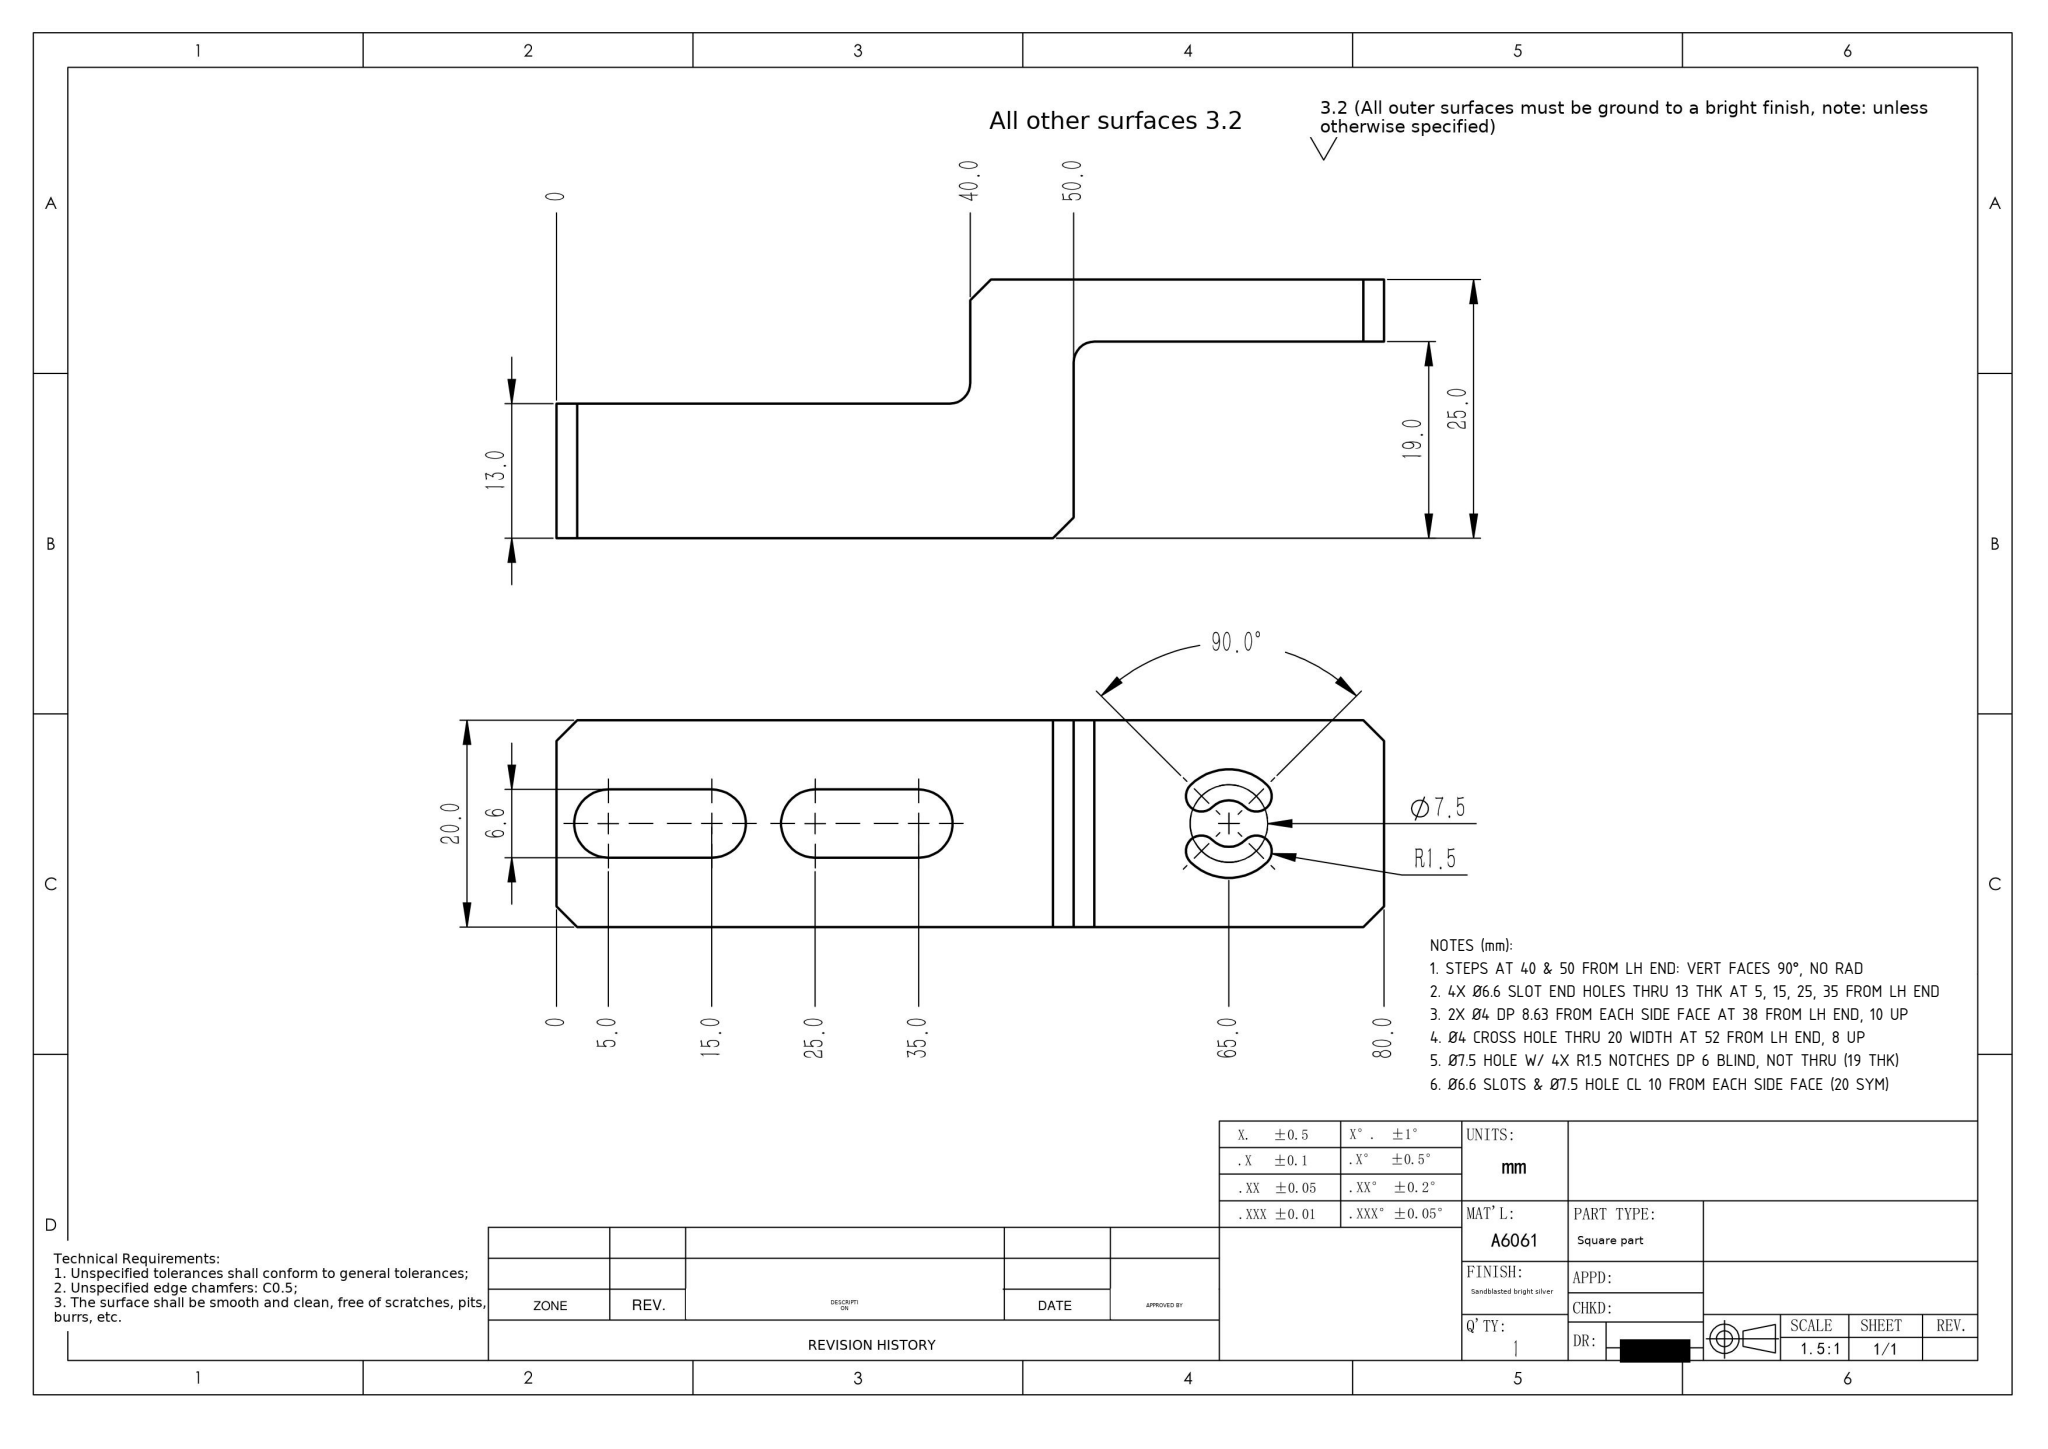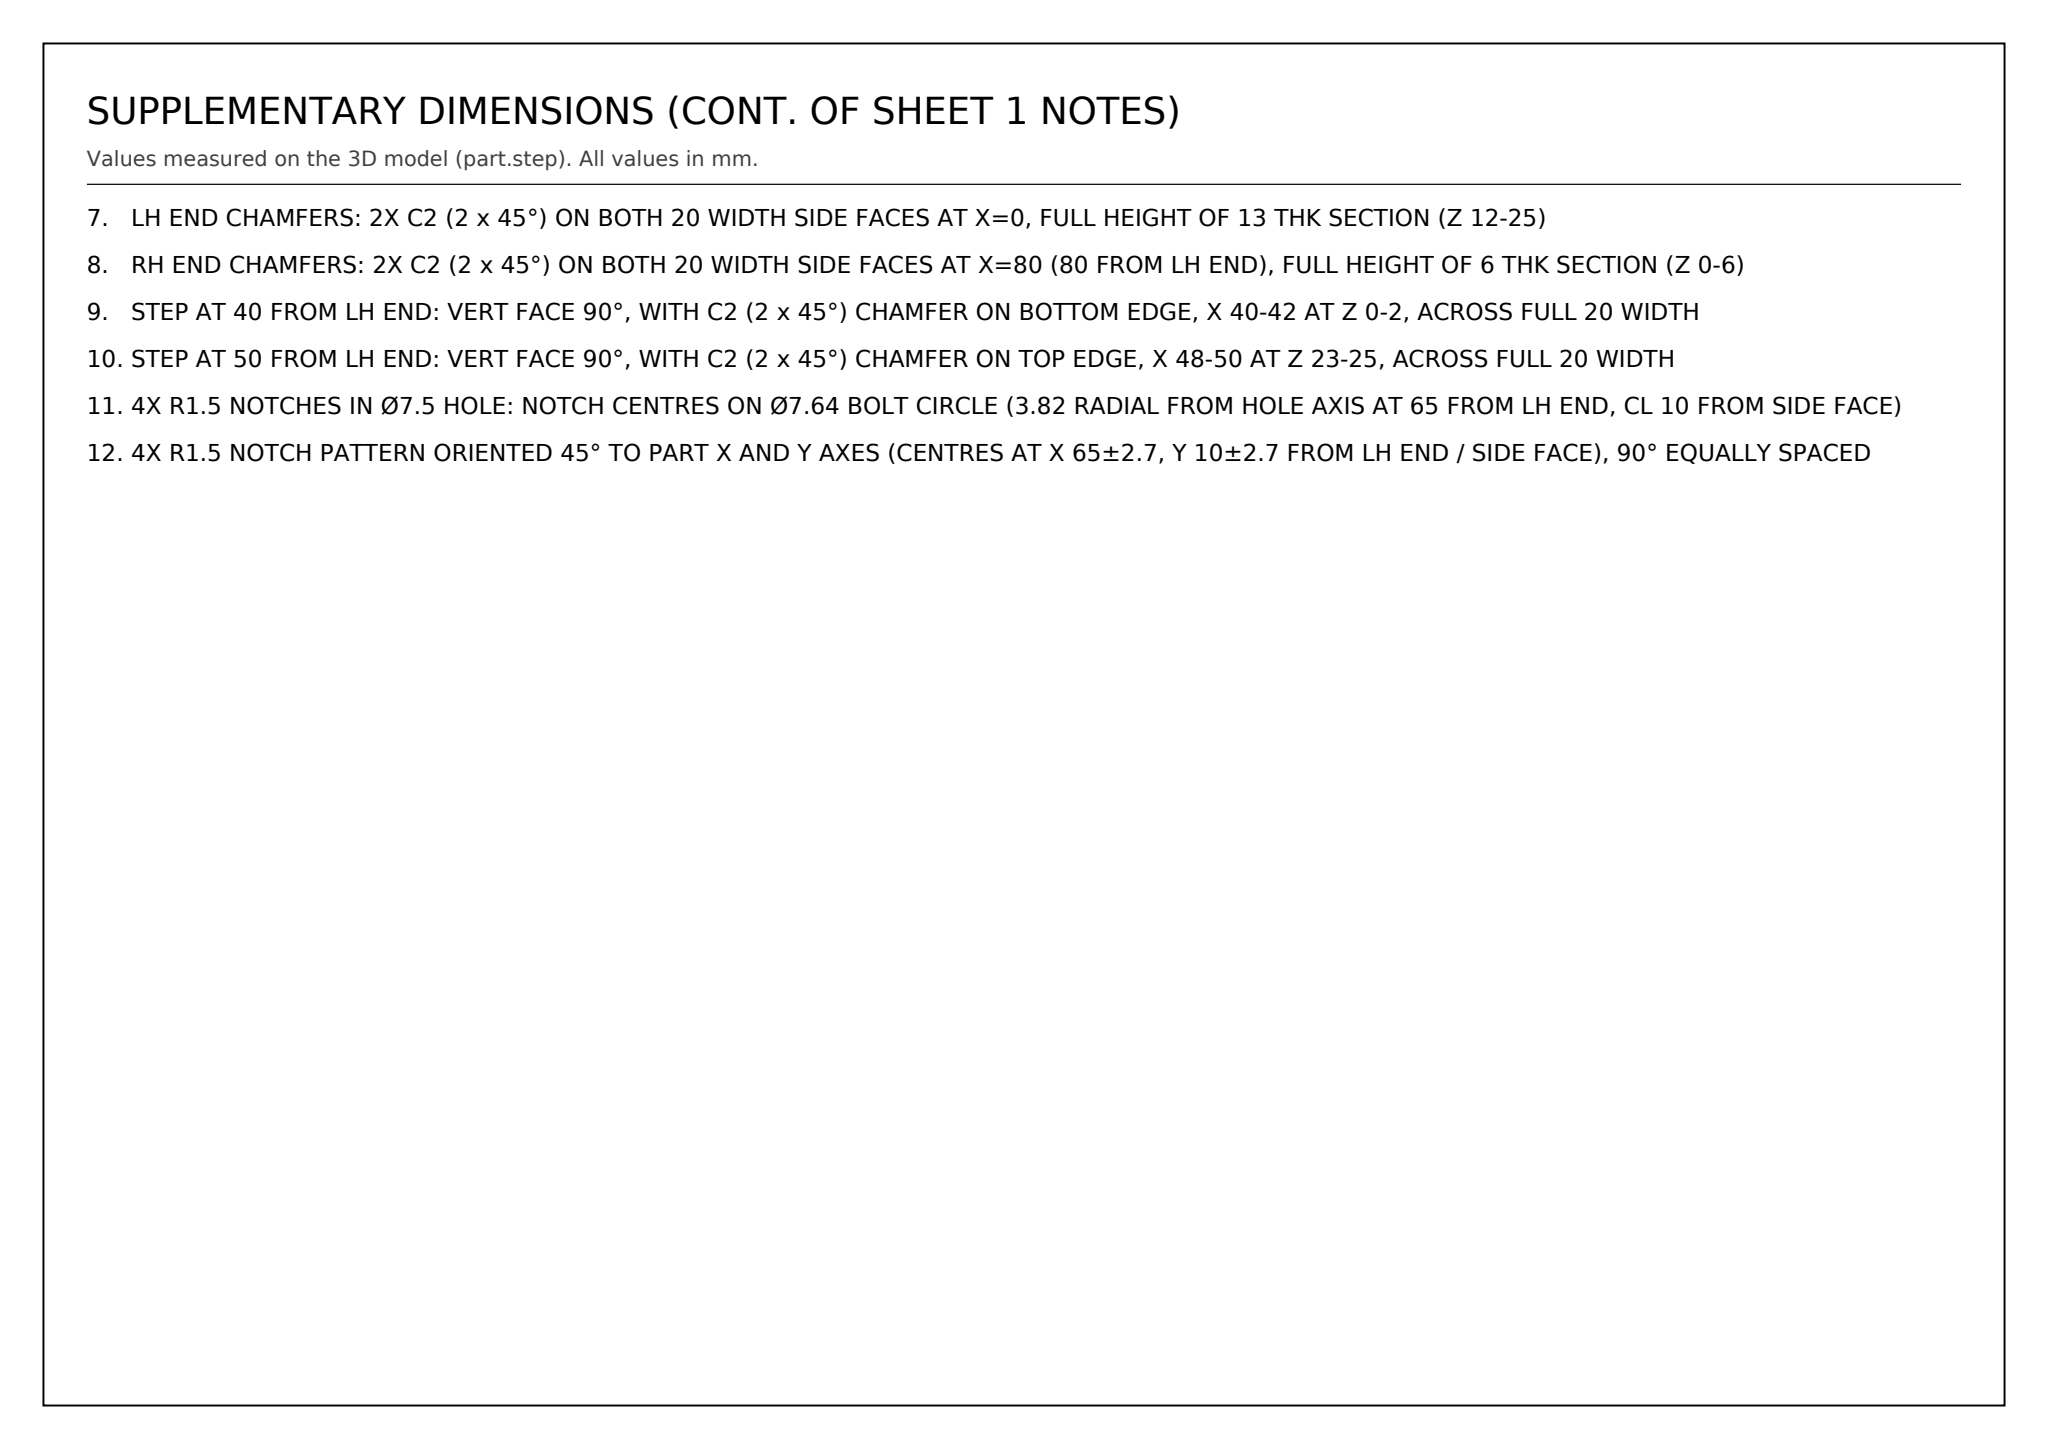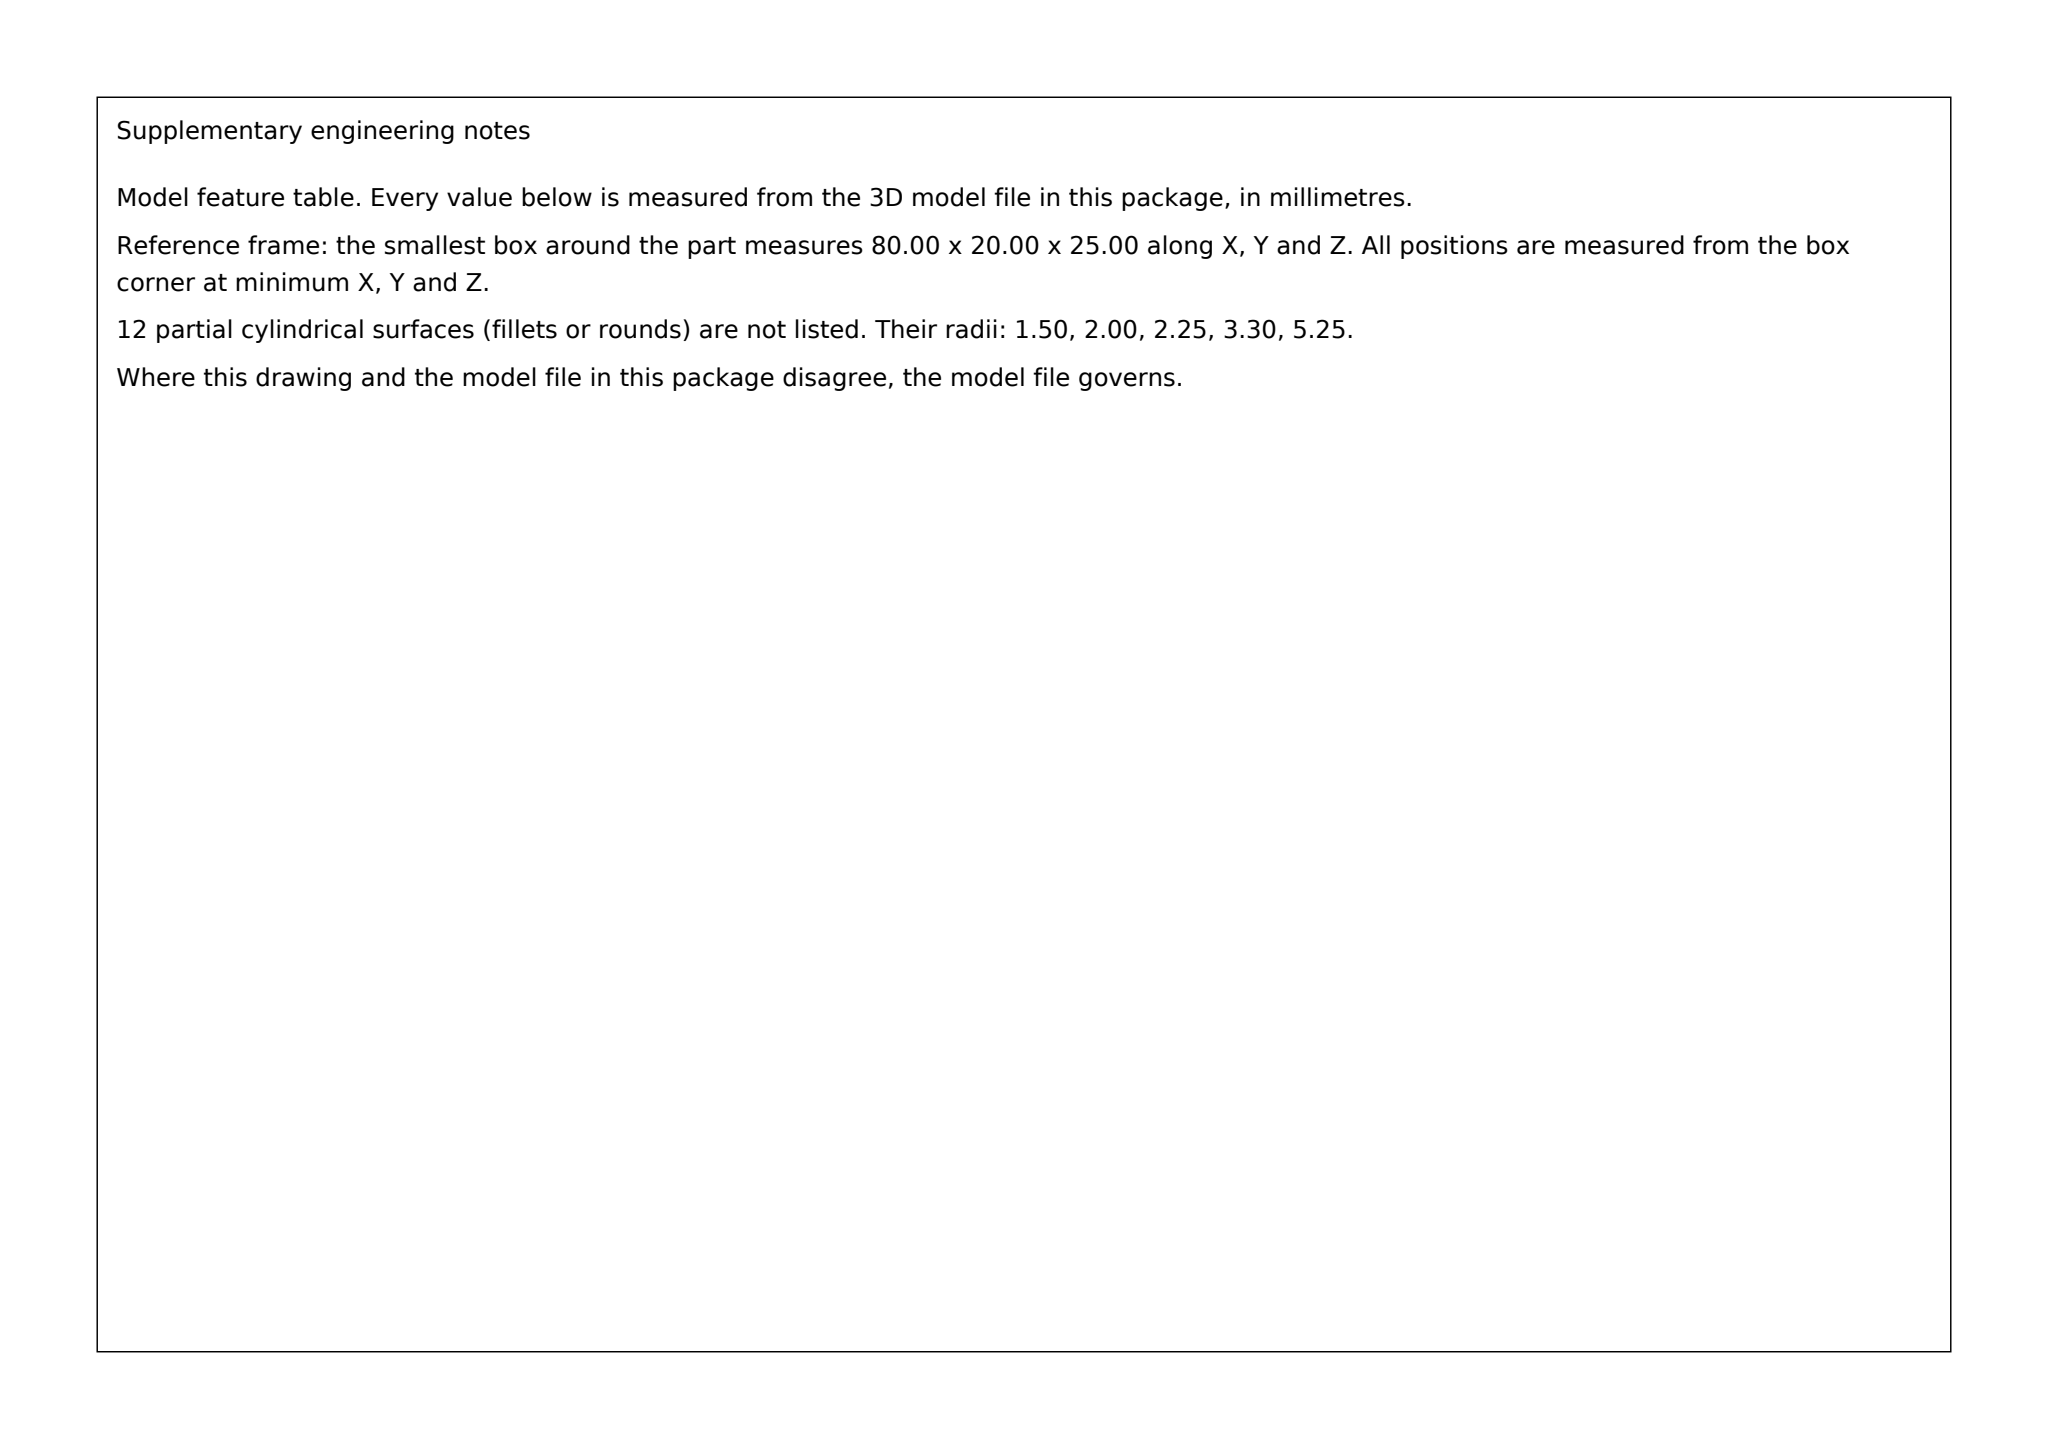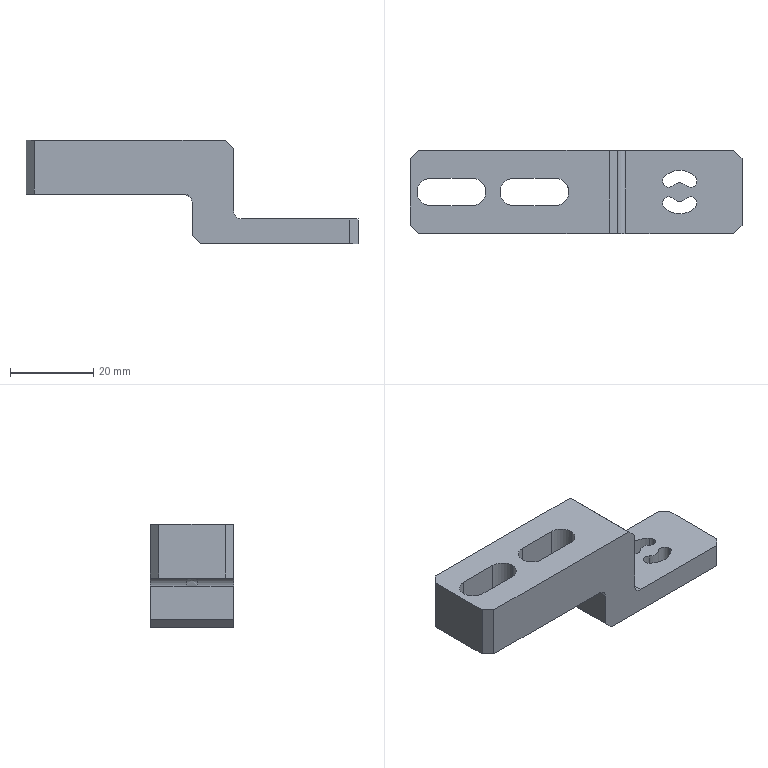Part | SolidWorks | mm | 1 solid | 40 faces | box 80 x 20 x 25 mm | volume 15976 mm3 | plane 20 | cylinder 19 | spline 1 | commonest cylinder face diameters 3 x6 6.6 x6 4 x3 4.5 x2 10.5 x2
Drawing notes:
STEPS AT 40 & 50 FROM LH END: VERT FACES 90°, NO RAD | from the solid: axis_planes x=40.0 and x=50.0 (planar faces normal to X); fillet_radii empty
4X Ø6.6 SLOT END HOLES THRU 13 THK AT 5, 15, 25, 35 FROM LH END | from the solid: cylinders dia 6.6, axis z, y=10.0, x=5/15/25/35, length 13.0 (full local thk)
2X Ø4 DP 8.63 FROM EACH SIDE FACE AT 38 FROM LH END, 10 UP | from the solid: cylinders [4.0,'y',[38.0,null,10.0],8.63] count 2, blind from each Y face
Ø4 CROSS HOLE THRU 20 WIDTH AT 52 FROM LH END, 8 UP | from the solid: cylinder dia 4.0, axis y, x=52, z=8, length 20.0 = full 20 width
Ø7.5 HOLE W/ 4X R1.5 NOTCHES DP 6 BLIND, NOT THRU (19 THK) | from the solid: cyls at [65,10] dia 10.5/4.5 len 6 + 4X dia 3.0 len 6 at (62.35/67.65, 7.35/12.65); z 6-25
Ø6.6 SLOTS & Ø7.5 HOLE CL 10 FROM EACH SIDE FACE (20 SYM) | from the solid: all 6.6 slot cyls and Ø7.5/Ø10.5 hole at y=10.0; bbox Y=20.0
LH END CHAMFERS: 2X C2 (2 x 45°) ON BOTH 20 WIDTH SIDE FACES AT X=0, FULL HEIGHT OF 13 THK SECTION (Z 12-25) | from the solid: inclined_planes angle_to_xyz_axes [45,45,90] bbox_from [0,0,12] and [0,18,12], size [2,2,13]
RH END CHAMFERS: 2X C2 (2 x 45°) ON BOTH 20 WIDTH SIDE FACES AT X=80 (80 FROM LH END), FULL HEIGHT OF 6 THK SECTION (Z 0-6) | from the solid: inclined_planes angle_to_xyz_axes [45,45,90] bbox_from [78,0,0] and [78,18,0], size [2,2,6]
STEP AT 40 FROM LH END: VERT FACE 90°, WITH C2 (2 x 45°) CHAMFER ON BOTTOM EDGE, X 40-42 AT Z 0-2, ACROSS FULL 20 WIDTH | from the solid: inclined_planes angle_to_xyz_axes [45,90,45] bbox_from [40,0,0], size [2,20,2]
STEP AT 50 FROM LH END: VERT FACE 90°, WITH C2 (2 x 45°) CHAMFER ON TOP EDGE, X 48-50 AT Z 23-25, ACROSS FULL 20 WIDTH | from the solid: inclined_planes angle_to_xyz_axes [45,90,45] bbox_from [48,0,23], size [2,20,2]
4X R1.5 NOTCHES IN Ø7.5 HOLE: NOTCH CENTRES ON Ø7.64 BOLT CIRCLE (3.82 RADIAL FROM HOLE AXIS AT 65 FROM LH END, CL 10 FROM SIDE FACE) | from the solid: cylinders: 4X dia 3.0 z-axis at (62.3,12.7),(62.3,7.3),(67.7,12.7),(67.7,7.3) vs Ø7.5 hole axis at (65.0,10.0) -> offset 2.7,2.7 = 3.82 radial
4X R1.5 NOTCH PATTERN ORIENTED 45° TO PART X AND Y AXES (CENTRES AT X 65±2.7, Y 10±2.7 FROM LH END / SIDE FACE), 90° EQUALLY SPACED | from the solid: cylinders: dia 3.0 notch centres at x 62.3/67.7 and y 7.3/12.7 about hole axis (65.0,10.0), equal ±2.7 offsets in x and y
build123d program:
from build123d import *

# Parameters (mm, degrees)
SKETCH1_W           = 80
SKETCH1_H           = 20
BOSS_EXTRUDE1_DEPTH = 25
SKETCH2_W           = 40
SKETCH2_H           = 20
CUT_EXTRUDE1_DEPTH  = 12
CUT_EXTRUDE2_DEPTH  = 85.41
CUT_EXTRUDE3_DEPTH  = 85.41
SKETCH5_W           = 30
SKETCH5_H           = 19
CUT_EXTRUDE4_DEPTH  = 87.168
CHAMFER1_SIZE       = 2
FILLET1_R           = 2


with BuildPart() as part:
    # Sketch1 → Boss-Extrude1 (new body)
    with BuildSketch(Plane.XY):
        with Locations((40, 0)):
            Rectangle(SKETCH1_W, SKETCH1_H)
    extrude(amount=BOSS_EXTRUDE1_DEPTH)

    # Sketch2 → Cut-Extrude1 (cut)
    with BuildSketch(Plane(origin=(0, 0, 0), x_dir=(-1, 0, 0), z_dir=(0, 0, -1))):
        with Locations((-20, 0)):
            Rectangle(SKETCH2_W, SKETCH2_H)
    extrude(amount=-CUT_EXTRUDE1_DEPTH, mode=Mode.SUBTRACT)

    # Sketch3 → Cut-Extrude2 (cut, through all)
    with BuildSketch(Plane.XY.offset(25)):
        with BuildLine():
            Line((5, 3.3), (15, 3.3))
            ThreePointArc((15, 3.3), (18.3, 0), (15, -3.3))
            Line((15, -3.3), (5, -3.3))
            ThreePointArc((5, -3.3), (1.7, 0), (5, 3.3))
        make_face()
        with BuildLine():
            Line((25, 3.3), (35, 3.3))
            ThreePointArc((35, 3.3), (38.3, 0), (35, -3.3))
            Line((35, -3.3), (25, -3.3))
            ThreePointArc((25, -3.3), (21.7, 0), (25, 3.3))
        make_face()
    extrude(amount=-CUT_EXTRUDE2_DEPTH, mode=Mode.SUBTRACT)

    # Sketch4 → Cut-Extrude3 (cut, through all)
    with BuildSketch(Plane.XY.offset(25)):
        with BuildLine():
            ThreePointArc((68.712, 3.712), (65, 5.25), (61.288, 3.712))
            ThreePointArc((61.288, 3.712), (61.288, 1.591), (63.409, 1.591))
            ThreePointArc((63.409, 1.591), (65, 2.25), (66.591, 1.591))
            ThreePointArc((66.591, 1.591), (68.712, 1.591), (68.712, 3.712))
        make_face()
        with BuildLine():
            ThreePointArc((68.712, -3.712), (65, -5.25), (61.288, -3.712))
            ThreePointArc((61.288, -3.712), (61.288, -1.591), (63.409, -1.591))
            ThreePointArc((63.409, -1.591), (65, -2.25), (66.591, -1.591))
            ThreePointArc((66.591, -1.591), (68.712, -1.591), (68.712, -3.712))
        make_face()
    extrude(amount=-CUT_EXTRUDE3_DEPTH, mode=Mode.SUBTRACT)

    # Sketch5 → Cut-Extrude4 (cut, through all)
    with BuildSketch(Plane(origin=(0, 10, 0), x_dir=(1, 0, 0), z_dir=(0, 1, 0))):
        with Locations((65, -15.5)):
            Rectangle(SKETCH5_W, SKETCH5_H)
    extrude(amount=-CUT_EXTRUDE4_DEPTH, mode=Mode.SUBTRACT)

    # Chamfer1
    chamfer1_edges = [part.edges().sort_by_distance(p)[0] for p in [
        (80, 10, 3),
        (80, -10, 3),
        (50, 0, 25),
        (40, 0, 0),
        (0, 10, 18.5),
        (0, -10, 18.5),
    ]]
    chamfer(chamfer1_edges, length=CHAMFER1_SIZE)

    # Fillet1
    fillet1_edges = [part.edges().sort_by_distance(p)[0] for p in [
        (50, 0, 6),
        (40, 0, 12),
    ]]
    fillet(fillet1_edges, radius=FILLET1_R)


solid = part.part